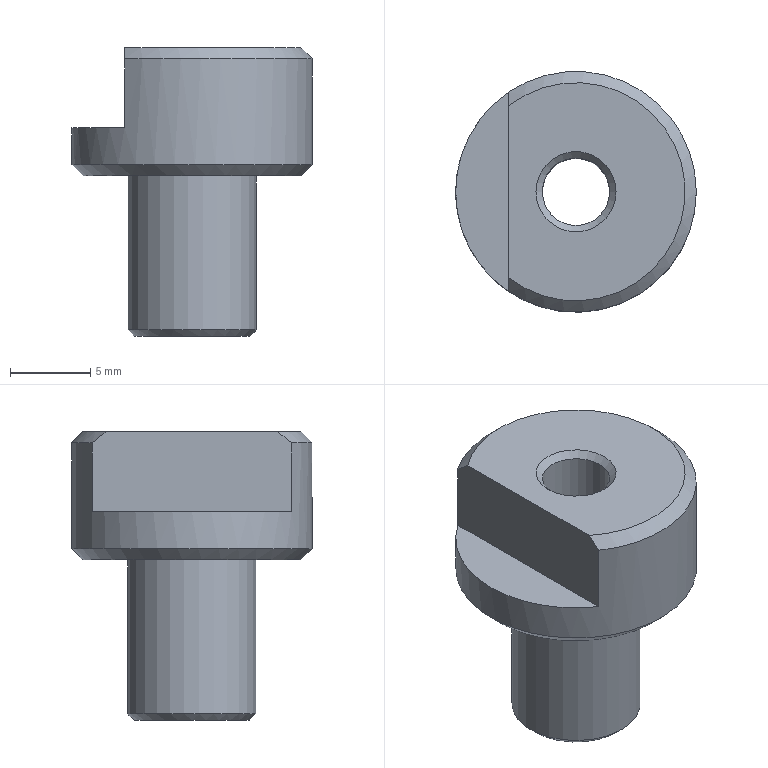Component | NX | DRILL_BUSHING_2 | 1 solid | 13 faces | box 15 x 15 x 18 mm | volume 1500 mm3 | plane 5 | cone 5 | cylinder 3 | commonest cylinder face diameters 8 x1 15 x1 4.2 x1
STEP:
#1=CARTESIAN_POINT('',(0.,0.,0.));
#2=DIRECTION('',(0.,0.,1.));
#3=DIRECTION('',(1.,0.,0.));
#4=AXIS2_PLACEMENT_3D('',#1,#2,#3);
#5=CARTESIAN_POINT('',(25.,0.,55.));
#6=VERTEX_POINT('',#5);
#7=CARTESIAN_POINT('',(22.5,0.,55.));
#8=DIRECTION('',(0.,0.,1.));
#9=DIRECTION('',(1.,0.,0.));
#10=AXIS2_PLACEMENT_3D('',#7,#8,#9);
#11=CIRCLE('',#10,2.5);
#12=CARTESIAN_POINT('',(22.5,0.,55.));
#13=DIRECTION('',(0.,0.,-1.));
#14=DIRECTION('',(1.,0.,0.));
#15=AXIS2_PLACEMENT_3D('',#12,#13,#14);
#16=PLANE('',#15);
#17=CARTESIAN_POINT('',(2.5,0.));
#18=CARTESIAN_POINT('',(2.5,-4.33));
#19=CARTESIAN_POINT('',(-1.25,-2.165));
#20=CARTESIAN_POINT('',(-5.,-0.));
#21=CARTESIAN_POINT('',(-1.25,2.165));
#22=CARTESIAN_POINT('',(2.5,4.33));
#23=CARTESIAN_POINT('',(2.5,0.));
#24=(BOUNDED_CURVE()B_SPLINE_CURVE(2,(#17,#18,#19,#20,#21,#22,#23),.UNSPECIFIED.,.T.,.F.)B_SPLINE_CURVE_WITH_KNOTS((1,2,2,2,2,1),(-2.094,0.,2.094,4.189,6.283,8.378),.UNSPECIFIED.)CURVE()GEOMETRIC_REPRESENTATION_ITEM()RATIONAL_B_SPLINE_CURVE((1.,0.5,1.,0.5,1.,0.5,1.))REPRESENTATION_ITEM(''));
#25=(GEOMETRIC_REPRESENTATION_CONTEXT(2)PARAMETRIC_REPRESENTATION_CONTEXT()REPRESENTATION_CONTEXT('',''));
#26=DEFINITIONAL_REPRESENTATION('',(#24),#25);
#27=PCURVE('',#16,#26);
#28=CARTESIAN_POINT('',(22.5,0.,55.4));
#29=DIRECTION('',(0.,0.,-1.));
#30=DIRECTION('',(1.,0.,0.));
#31=AXIS2_PLACEMENT_3D('',#28,#29,#30);
#32=CONICAL_SURFACE('',#31,2.1,0.7854);
#33=CARTESIAN_POINT('',(6.283,0.4));
#34=DIRECTION('',(-1.,0.));
#35=VECTOR('',#34,1.);
#36=LINE('',#33,#35);
#37=(GEOMETRIC_REPRESENTATION_CONTEXT(2)PARAMETRIC_REPRESENTATION_CONTEXT()REPRESENTATION_CONTEXT('',''));
#38=DEFINITIONAL_REPRESENTATION('',(#36),#37);
#39=PCURVE('',#32,#38);
#40=SURFACE_CURVE('',#11,(#27,#39),.PCURVE_S1.);
#41=EDGE_CURVE('',#6,#6,#40,.T.);
#42=ORIENTED_EDGE('',*,*,#41,.T.);
#43=EDGE_LOOP('',(#42));
#44=FACE_BOUND('',#43,.T.);
#45=CARTESIAN_POINT('',(26.1,0.,55.));
#46=VERTEX_POINT('',#45);
#47=CARTESIAN_POINT('',(22.5,0.,55.));
#48=DIRECTION('',(0.,0.,-1.));
#49=DIRECTION('',(1.,0.,0.));
#50=AXIS2_PLACEMENT_3D('',#47,#48,#49);
#51=CIRCLE('',#50,3.6);
#52=CARTESIAN_POINT('',(0.,0.));
#53=DIRECTION('',(1.,0.));
#54=AXIS2_PLACEMENT_2D('',#52,#53);
#55=CIRCLE('',#54,3.6);
#56=(GEOMETRIC_REPRESENTATION_CONTEXT(2)PARAMETRIC_REPRESENTATION_CONTEXT()REPRESENTATION_CONTEXT('',''));
#57=DEFINITIONAL_REPRESENTATION('',(#55),#56);
#58=PCURVE('',#16,#57);
#59=CARTESIAN_POINT('',(22.5,0.,55.4));
#60=DIRECTION('',(0.,0.,1.));
#61=DIRECTION('',(-1.,0.,0.));
#62=AXIS2_PLACEMENT_3D('',#59,#60,#61);
#63=CONICAL_SURFACE('',#62,4.,0.7854);
#64=CARTESIAN_POINT('',(9.425,-0.4));
#65=DIRECTION('',(-1.,0.));
#66=VECTOR('',#65,1.);
#67=LINE('',#64,#66);
#68=(GEOMETRIC_REPRESENTATION_CONTEXT(2)PARAMETRIC_REPRESENTATION_CONTEXT()REPRESENTATION_CONTEXT('',''));
#69=DEFINITIONAL_REPRESENTATION('',(#67),#68);
#70=PCURVE('',#63,#69);
#71=SURFACE_CURVE('',#51,(#58,#70),.PCURVE_S1.);
#72=EDGE_CURVE('',#46,#46,#71,.T.);
#73=ORIENTED_EDGE('',*,*,#72,.T.);
#74=EDGE_LOOP('',(#73));
#75=FACE_BOUND('',#74,.T.);
#76=ADVANCED_FACE('',(#44,#75),#16,.T.);
#77=CARTESIAN_POINT('',(26.5,0.,55.4));
#78=VERTEX_POINT('',#77);
#79=CARTESIAN_POINT('',(22.5,0.,55.4));
#80=DIRECTION('',(0.,0.,1.));
#81=DIRECTION('',(1.,0.,0.));
#82=AXIS2_PLACEMENT_3D('',#79,#80,#81);
#83=CIRCLE('',#82,4.);
#84=CARTESIAN_POINT('',(22.5,0.,55.));
#85=DIRECTION('',(0.,0.,1.));
#86=DIRECTION('',(-1.,0.,0.));
#87=AXIS2_PLACEMENT_3D('',#84,#85,#86);
#88=CYLINDRICAL_SURFACE('',#87,4.);
#89=CARTESIAN_POINT('',(3.142,0.4));
#90=DIRECTION('',(1.,0.));
#91=VECTOR('',#90,1.);
#92=LINE('',#89,#91);
#93=(GEOMETRIC_REPRESENTATION_CONTEXT(2)PARAMETRIC_REPRESENTATION_CONTEXT()REPRESENTATION_CONTEXT('',''));
#94=DEFINITIONAL_REPRESENTATION('',(#92),#93);
#95=PCURVE('',#88,#94);
#96=CARTESIAN_POINT('',(3.142,0.));
#97=DIRECTION('',(1.,0.));
#98=VECTOR('',#97,1.);
#99=LINE('',#96,#98);
#100=(GEOMETRIC_REPRESENTATION_CONTEXT(2)PARAMETRIC_REPRESENTATION_CONTEXT()REPRESENTATION_CONTEXT('',''));
#101=DEFINITIONAL_REPRESENTATION('',(#99),#100);
#102=PCURVE('',#63,#101);
#103=SURFACE_CURVE('',#83,(#95,#102),.PCURVE_S1.);
#104=EDGE_CURVE('',#78,#78,#103,.T.);
#105=ORIENTED_EDGE('',*,*,#104,.T.);
#106=CARTESIAN_POINT('',(26.5,0.,65.));
#107=VERTEX_POINT('',#106);
#108=CARTESIAN_POINT('',(26.5,0.,55.4));
#109=CARTESIAN_POINT('',(26.5,0.,65.));
#110=B_SPLINE_CURVE_WITH_KNOTS('',1,(#108,#109),.UNSPECIFIED.,.F.,.F.,(2,2),(0.4,10.),.PIECEWISE_BEZIER_KNOTS.);
#111=CARTESIAN_POINT('',(9.425,0.));
#112=DIRECTION('',(0.,1.));
#113=VECTOR('',#112,1.);
#114=LINE('',#111,#113);
#115=(GEOMETRIC_REPRESENTATION_CONTEXT(2)PARAMETRIC_REPRESENTATION_CONTEXT()REPRESENTATION_CONTEXT('',''));
#116=DEFINITIONAL_REPRESENTATION('',(#114),#115);
#117=PCURVE('',#88,#116);
#118=CARTESIAN_POINT('',(3.142,0.));
#119=DIRECTION('',(0.,1.));
#120=VECTOR('',#119,1.);
#121=LINE('',#118,#120);
#122=(GEOMETRIC_REPRESENTATION_CONTEXT(2)PARAMETRIC_REPRESENTATION_CONTEXT()REPRESENTATION_CONTEXT('',''));
#123=DEFINITIONAL_REPRESENTATION('',(#121),#122);
#124=PCURVE('',#88,#123);
#125=SEAM_CURVE('',#110,(#117,#124),.PCURVE_S1.);
#126=EDGE_CURVE('',#78,#107,#125,.T.);
#127=ORIENTED_EDGE('',*,*,#126,.T.);
#128=CARTESIAN_POINT('',(22.5,0.,65.));
#129=DIRECTION('',(0.,0.,1.));
#130=DIRECTION('',(1.,0.,0.));
#131=AXIS2_PLACEMENT_3D('',#128,#129,#130);
#132=CIRCLE('',#131,4.);
#133=CARTESIAN_POINT('',(3.142,10.));
#134=DIRECTION('',(1.,0.));
#135=VECTOR('',#134,1.);
#136=LINE('',#133,#135);
#137=(GEOMETRIC_REPRESENTATION_CONTEXT(2)PARAMETRIC_REPRESENTATION_CONTEXT()REPRESENTATION_CONTEXT('',''));
#138=DEFINITIONAL_REPRESENTATION('',(#136),#137);
#139=PCURVE('',#88,#138);
#140=CARTESIAN_POINT('',(22.5,0.,65.));
#141=DIRECTION('',(0.,0.,-1.));
#142=DIRECTION('',(1.,0.,0.));
#143=AXIS2_PLACEMENT_3D('',#140,#141,#142);
#144=PLANE('',#143);
#145=CARTESIAN_POINT('',(4.,0.));
#146=CARTESIAN_POINT('',(4.,-6.928));
#147=CARTESIAN_POINT('',(-2.,-3.464));
#148=CARTESIAN_POINT('',(-8.,-0.));
#149=CARTESIAN_POINT('',(-2.,3.464));
#150=CARTESIAN_POINT('',(4.,6.928));
#151=CARTESIAN_POINT('',(4.,0.));
#152=(BOUNDED_CURVE()B_SPLINE_CURVE(2,(#145,#146,#147,#148,#149,#150,#151),.UNSPECIFIED.,.T.,.F.)B_SPLINE_CURVE_WITH_KNOTS((1,2,2,2,2,1),(-2.094,0.,2.094,4.189,6.283,8.378),.UNSPECIFIED.)CURVE()GEOMETRIC_REPRESENTATION_ITEM()RATIONAL_B_SPLINE_CURVE((1.,0.5,1.,0.5,1.,0.5,1.))REPRESENTATION_ITEM(''));
#153=(GEOMETRIC_REPRESENTATION_CONTEXT(2)PARAMETRIC_REPRESENTATION_CONTEXT()REPRESENTATION_CONTEXT('',''));
#154=DEFINITIONAL_REPRESENTATION('',(#152),#153);
#155=PCURVE('',#144,#154);
#156=SURFACE_CURVE('',#132,(#139,#155),.PCURVE_S1.);
#157=EDGE_CURVE('',#107,#107,#156,.T.);
#158=ORIENTED_EDGE('',*,*,#157,.F.);
#159=ORIENTED_EDGE('',*,*,#126,.F.);
#160=EDGE_LOOP('',(#105,#127,#158,#159));
#161=FACE_BOUND('',#160,.T.);
#162=ADVANCED_FACE('',(#161),#88,.T.);
#163=CARTESIAN_POINT('',(20.,0.,73.));
#164=VERTEX_POINT('',#163);
#165=CARTESIAN_POINT('',(22.5,0.,73.));
#166=DIRECTION('',(0.,0.,-1.));
#167=DIRECTION('',(-1.,0.,0.));
#168=AXIS2_PLACEMENT_3D('',#165,#166,#167);
#169=CIRCLE('',#168,2.5);
#170=CARTESIAN_POINT('',(22.5,0.,73.));
#171=DIRECTION('',(0.,0.,1.));
#172=DIRECTION('',(-1.,0.,0.));
#173=AXIS2_PLACEMENT_3D('',#170,#171,#172);
#174=PLANE('',#173);
#175=CARTESIAN_POINT('',(2.5,0.));
#176=CARTESIAN_POINT('',(2.5,-4.33));
#177=CARTESIAN_POINT('',(-1.25,-2.165));
#178=CARTESIAN_POINT('',(-5.,-0.));
#179=CARTESIAN_POINT('',(-1.25,2.165));
#180=CARTESIAN_POINT('',(2.5,4.33));
#181=CARTESIAN_POINT('',(2.5,0.));
#182=(BOUNDED_CURVE()B_SPLINE_CURVE(2,(#175,#176,#177,#178,#179,#180,#181),.UNSPECIFIED.,.T.,.F.)B_SPLINE_CURVE_WITH_KNOTS((1,2,2,2,2,1),(-2.094,0.,2.094,4.189,6.283,8.378),.UNSPECIFIED.)CURVE()GEOMETRIC_REPRESENTATION_ITEM()RATIONAL_B_SPLINE_CURVE((1.,0.5,1.,0.5,1.,0.5,1.))REPRESENTATION_ITEM(''));
#183=(GEOMETRIC_REPRESENTATION_CONTEXT(2)PARAMETRIC_REPRESENTATION_CONTEXT()REPRESENTATION_CONTEXT('',''));
#184=DEFINITIONAL_REPRESENTATION('',(#182),#183);
#185=PCURVE('',#174,#184);
#186=CARTESIAN_POINT('',(22.5,0.,73.));
#187=DIRECTION('',(0.,0.,1.));
#188=DIRECTION('',(-1.,0.,0.));
#189=AXIS2_PLACEMENT_3D('',#186,#187,#188);
#190=CONICAL_SURFACE('',#189,2.5,0.7854);
#191=CARTESIAN_POINT('',(6.283,0.));
#192=DIRECTION('',(-1.,0.));
#193=VECTOR('',#192,1.);
#194=LINE('',#191,#193);
#195=(GEOMETRIC_REPRESENTATION_CONTEXT(2)PARAMETRIC_REPRESENTATION_CONTEXT()REPRESENTATION_CONTEXT('',''));
#196=DEFINITIONAL_REPRESENTATION('',(#194),#195);
#197=PCURVE('',#190,#196);
#198=SURFACE_CURVE('',#169,(#185,#197),.PCURVE_S1.);
#199=EDGE_CURVE('',#164,#164,#198,.T.);
#200=ORIENTED_EDGE('',*,*,#199,.T.);
#201=EDGE_LOOP('',(#200));
#202=FACE_BOUND('',#201,.T.);
#203=CARTESIAN_POINT('',(18.3,-5.348,73.));
#204=VERTEX_POINT('',#203);
#205=CARTESIAN_POINT('',(18.3,5.348,73.));
#206=VERTEX_POINT('',#205);
#207=CARTESIAN_POINT('',(18.3,-7.102,73.));
#208=DIRECTION('',(-0.,1.,0.));
#209=VECTOR('',#208,1.);
#210=LINE('',#207,#209);
#211=CARTESIAN_POINT('',(4.2,7.102));
#212=DIRECTION('',(0.,-1.));
#213=VECTOR('',#212,1.);
#214=LINE('',#211,#213);
#215=(GEOMETRIC_REPRESENTATION_CONTEXT(2)PARAMETRIC_REPRESENTATION_CONTEXT()REPRESENTATION_CONTEXT('',''));
#216=DEFINITIONAL_REPRESENTATION('',(#214),#215);
#217=PCURVE('',#174,#216);
#218=CARTESIAN_POINT('',(18.3,-7.102,68.));
#219=DIRECTION('',(1.,0.,0.));
#220=DIRECTION('',(-0.,1.,0.));
#221=AXIS2_PLACEMENT_3D('',#218,#219,#220);
#222=PLANE('',#221);
#223=CARTESIAN_POINT('',(0.,5.));
#224=DIRECTION('',(1.,0.));
#225=VECTOR('',#224,1.);
#226=LINE('',#223,#225);
#227=(GEOMETRIC_REPRESENTATION_CONTEXT(2)PARAMETRIC_REPRESENTATION_CONTEXT()REPRESENTATION_CONTEXT('',''));
#228=DEFINITIONAL_REPRESENTATION('',(#226),#227);
#229=PCURVE('',#222,#228);
#230=SURFACE_CURVE('',#210,(#217,#229),.PCURVE_S1.);
#231=EDGE_CURVE('',#204,#206,#230,.T.);
#232=ORIENTED_EDGE('',*,*,#231,.F.);
#233=CARTESIAN_POINT('',(22.5,0.,73.));
#234=DIRECTION('',(0.,0.,1.));
#235=DIRECTION('',(-1.,0.,0.));
#236=AXIS2_PLACEMENT_3D('',#233,#234,#235);
#237=CIRCLE('',#236,6.8);
#238=CARTESIAN_POINT('',(0.,0.));
#239=DIRECTION('',(1.,0.));
#240=AXIS2_PLACEMENT_2D('',#238,#239);
#241=CIRCLE('',#240,6.8);
#242=(GEOMETRIC_REPRESENTATION_CONTEXT(2)PARAMETRIC_REPRESENTATION_CONTEXT()REPRESENTATION_CONTEXT('',''));
#243=DEFINITIONAL_REPRESENTATION('',(#241),#242);
#244=PCURVE('',#174,#243);
#245=CARTESIAN_POINT('',(22.5,0.,72.3));
#246=DIRECTION('',(0.,0.,-1.));
#247=DIRECTION('',(1.,0.,0.));
#248=AXIS2_PLACEMENT_3D('',#245,#246,#247);
#249=CONICAL_SURFACE('',#248,7.5,0.7854);
#250=CARTESIAN_POINT('',(9.425,-0.7));
#251=DIRECTION('',(-1.,-0.));
#252=VECTOR('',#251,1.);
#253=LINE('',#250,#252);
#254=(GEOMETRIC_REPRESENTATION_CONTEXT(2)PARAMETRIC_REPRESENTATION_CONTEXT()REPRESENTATION_CONTEXT('',''));
#255=DEFINITIONAL_REPRESENTATION('',(#253),#254);
#256=PCURVE('',#249,#255);
#257=SURFACE_CURVE('',#237,(#244,#256),.PCURVE_S1.);
#258=EDGE_CURVE('',#204,#206,#257,.T.);
#259=ORIENTED_EDGE('',*,*,#258,.T.);
#260=EDGE_LOOP('',(#232,#259));
#261=FACE_BOUND('',#260,.T.);
#262=ADVANCED_FACE('',(#202,#261),#174,.T.);
#263=CARTESIAN_POINT('',(29.3,0.,65.));
#264=VERTEX_POINT('',#263);
#265=CARTESIAN_POINT('',(22.5,0.,65.));
#266=DIRECTION('',(0.,0.,-1.));
#267=DIRECTION('',(1.,0.,0.));
#268=AXIS2_PLACEMENT_3D('',#265,#266,#267);
#269=CIRCLE('',#268,6.8);
#270=CARTESIAN_POINT('',(0.,0.));
#271=DIRECTION('',(1.,0.));
#272=AXIS2_PLACEMENT_2D('',#270,#271);
#273=CIRCLE('',#272,6.8);
#274=(GEOMETRIC_REPRESENTATION_CONTEXT(2)PARAMETRIC_REPRESENTATION_CONTEXT()REPRESENTATION_CONTEXT('',''));
#275=DEFINITIONAL_REPRESENTATION('',(#273),#274);
#276=PCURVE('',#144,#275);
#277=CARTESIAN_POINT('',(22.5,0.,65.7));
#278=DIRECTION('',(0.,0.,1.));
#279=DIRECTION('',(-1.,0.,0.));
#280=AXIS2_PLACEMENT_3D('',#277,#278,#279);
#281=CONICAL_SURFACE('',#280,7.5,0.7854);
#282=CARTESIAN_POINT('',(9.425,-0.7));
#283=DIRECTION('',(-1.,0.));
#284=VECTOR('',#283,1.);
#285=LINE('',#282,#284);
#286=(GEOMETRIC_REPRESENTATION_CONTEXT(2)PARAMETRIC_REPRESENTATION_CONTEXT()REPRESENTATION_CONTEXT('',''));
#287=DEFINITIONAL_REPRESENTATION('',(#285),#286);
#288=PCURVE('',#281,#287);
#289=SURFACE_CURVE('',#269,(#276,#288),.PCURVE_S1.);
#290=EDGE_CURVE('',#264,#264,#289,.T.);
#291=ORIENTED_EDGE('',*,*,#290,.T.);
#292=EDGE_LOOP('',(#291));
#293=FACE_BOUND('',#292,.T.);
#294=ORIENTED_EDGE('',*,*,#157,.T.);
#295=EDGE_LOOP('',(#294));
#296=FACE_BOUND('',#295,.T.);
#297=ADVANCED_FACE('',(#293,#296),#144,.T.);
#298=CARTESIAN_POINT('',(30.,0.,65.7));
#299=VERTEX_POINT('',#298);
#300=CARTESIAN_POINT('',(18.3,6.214,65.7));
#301=VERTEX_POINT('',#300);
#302=CARTESIAN_POINT('',(22.5,0.,65.7));
#303=DIRECTION('',(0.,0.,1.));
#304=DIRECTION('',(1.,0.,0.));
#305=AXIS2_PLACEMENT_3D('',#302,#303,#304);
#306=CIRCLE('',#305,7.5);
#307=CARTESIAN_POINT('',(22.5,0.,65.));
#308=DIRECTION('',(0.,0.,1.));
#309=DIRECTION('',(-1.,0.,0.));
#310=AXIS2_PLACEMENT_3D('',#307,#308,#309);
#311=CYLINDRICAL_SURFACE('',#310,7.5);
#312=CARTESIAN_POINT('',(9.425,0.7));
#313=DIRECTION('',(1.,0.));
#314=VECTOR('',#313,1.);
#315=LINE('',#312,#314);
#316=(GEOMETRIC_REPRESENTATION_CONTEXT(2)PARAMETRIC_REPRESENTATION_CONTEXT()REPRESENTATION_CONTEXT('',''));
#317=DEFINITIONAL_REPRESENTATION('',(#315),#316);
#318=PCURVE('',#311,#317);
#319=CARTESIAN_POINT('',(3.142,0.));
#320=DIRECTION('',(1.,0.));
#321=VECTOR('',#320,1.);
#322=LINE('',#319,#321);
#323=(GEOMETRIC_REPRESENTATION_CONTEXT(2)PARAMETRIC_REPRESENTATION_CONTEXT()REPRESENTATION_CONTEXT('',''));
#324=DEFINITIONAL_REPRESENTATION('',(#322),#323);
#325=PCURVE('',#281,#324);
#326=SURFACE_CURVE('',#306,(#318,#325),.PCURVE_S1.);
#327=EDGE_CURVE('',#299,#301,#326,.T.);
#328=ORIENTED_EDGE('',*,*,#327,.T.);
#329=CARTESIAN_POINT('',(18.3,6.214,68.));
#330=VERTEX_POINT('',#329);
#331=CARTESIAN_POINT('',(18.3,6.214,65.7));
#332=CARTESIAN_POINT('',(18.3,6.214,68.));
#333=B_SPLINE_CURVE_WITH_KNOTS('',1,(#331,#332),.UNSPECIFIED.,.F.,.F.,(2,2),(0.7,3.),.PIECEWISE_BEZIER_KNOTS.);
#334=CARTESIAN_POINT('',(11.59,0.));
#335=DIRECTION('',(0.,1.));
#336=VECTOR('',#335,1.);
#337=LINE('',#334,#336);
#338=(GEOMETRIC_REPRESENTATION_CONTEXT(2)PARAMETRIC_REPRESENTATION_CONTEXT()REPRESENTATION_CONTEXT('',''));
#339=DEFINITIONAL_REPRESENTATION('',(#337),#338);
#340=PCURVE('',#311,#339);
#341=CARTESIAN_POINT('',(5.307,0.));
#342=DIRECTION('',(0.,1.));
#343=VECTOR('',#342,1.);
#344=LINE('',#341,#343);
#345=(GEOMETRIC_REPRESENTATION_CONTEXT(2)PARAMETRIC_REPRESENTATION_CONTEXT()REPRESENTATION_CONTEXT('',''));
#346=DEFINITIONAL_REPRESENTATION('',(#344),#345);
#347=PCURVE('',#311,#346);
#348=SEAM_CURVE('',#333,(#340,#347),.PCURVE_S1.);
#349=EDGE_CURVE('',#301,#330,#348,.T.);
#350=ORIENTED_EDGE('',*,*,#349,.T.);
#351=CARTESIAN_POINT('',(18.3,6.214,72.3));
#352=VERTEX_POINT('',#351);
#353=CARTESIAN_POINT('',(18.3,6.214,65.));
#354=DIRECTION('',(0.,0.,-1.));
#355=VECTOR('',#354,1.);
#356=LINE('',#353,#355);
#357=CARTESIAN_POINT('',(11.59,0.));
#358=DIRECTION('',(0.,-1.));
#359=VECTOR('',#358,1.);
#360=LINE('',#357,#359);
#361=(GEOMETRIC_REPRESENTATION_CONTEXT(2)PARAMETRIC_REPRESENTATION_CONTEXT()REPRESENTATION_CONTEXT('',''));
#362=DEFINITIONAL_REPRESENTATION('',(#360),#361);
#363=PCURVE('',#311,#362);
#364=CARTESIAN_POINT('',(13.316,-3.));
#365=DIRECTION('',(0.,-1.));
#366=VECTOR('',#365,1.);
#367=LINE('',#364,#366);
#368=(GEOMETRIC_REPRESENTATION_CONTEXT(2)PARAMETRIC_REPRESENTATION_CONTEXT()REPRESENTATION_CONTEXT('',''));
#369=DEFINITIONAL_REPRESENTATION('',(#367),#368);
#370=PCURVE('',#222,#369);
#371=SURFACE_CURVE('',#356,(#363,#370),.PCURVE_S1.);
#372=EDGE_CURVE('',#352,#330,#371,.T.);
#373=ORIENTED_EDGE('',*,*,#372,.F.);
#374=CARTESIAN_POINT('',(18.3,-6.214,72.3));
#375=VERTEX_POINT('',#374);
#376=CARTESIAN_POINT('',(22.5,0.,72.3));
#377=DIRECTION('',(0.,0.,-1.));
#378=DIRECTION('',(-1.,0.,0.));
#379=AXIS2_PLACEMENT_3D('',#376,#377,#378);
#380=CIRCLE('',#379,7.5);
#381=CARTESIAN_POINT('',(12.566,7.3));
#382=DIRECTION('',(-1.,0.));
#383=VECTOR('',#382,1.);
#384=LINE('',#381,#383);
#385=(GEOMETRIC_REPRESENTATION_CONTEXT(2)PARAMETRIC_REPRESENTATION_CONTEXT()REPRESENTATION_CONTEXT('',''));
#386=DEFINITIONAL_REPRESENTATION('',(#384),#385);
#387=PCURVE('',#311,#386);
#388=CARTESIAN_POINT('',(3.142,0.));
#389=DIRECTION('',(1.,-0.));
#390=VECTOR('',#389,1.);
#391=LINE('',#388,#390);
#392=(GEOMETRIC_REPRESENTATION_CONTEXT(2)PARAMETRIC_REPRESENTATION_CONTEXT()REPRESENTATION_CONTEXT('',''));
#393=DEFINITIONAL_REPRESENTATION('',(#391),#392);
#394=PCURVE('',#249,#393);
#395=SURFACE_CURVE('',#380,(#387,#394),.PCURVE_S1.);
#396=EDGE_CURVE('',#352,#375,#395,.T.);
#397=ORIENTED_EDGE('',*,*,#396,.T.);
#398=CARTESIAN_POINT('',(18.3,-6.214,68.));
#399=VERTEX_POINT('',#398);
#400=CARTESIAN_POINT('',(18.3,-6.214,65.));
#401=DIRECTION('',(0.,0.,1.));
#402=VECTOR('',#401,1.);
#403=LINE('',#400,#402);
#404=CARTESIAN_POINT('',(7.26,0.));
#405=DIRECTION('',(0.,1.));
#406=VECTOR('',#405,1.);
#407=LINE('',#404,#406);
#408=(GEOMETRIC_REPRESENTATION_CONTEXT(2)PARAMETRIC_REPRESENTATION_CONTEXT()REPRESENTATION_CONTEXT('',''));
#409=DEFINITIONAL_REPRESENTATION('',(#407),#408);
#410=PCURVE('',#311,#409);
#411=CARTESIAN_POINT('',(0.8883,-3.));
#412=DIRECTION('',(0.,1.));
#413=VECTOR('',#412,1.);
#414=LINE('',#411,#413);
#415=(GEOMETRIC_REPRESENTATION_CONTEXT(2)PARAMETRIC_REPRESENTATION_CONTEXT()REPRESENTATION_CONTEXT('',''));
#416=DEFINITIONAL_REPRESENTATION('',(#414),#415);
#417=PCURVE('',#222,#416);
#418=SURFACE_CURVE('',#403,(#410,#417),.PCURVE_S1.);
#419=EDGE_CURVE('',#399,#375,#418,.T.);
#420=ORIENTED_EDGE('',*,*,#419,.F.);
#421=CARTESIAN_POINT('',(22.5,0.,68.));
#422=DIRECTION('',(0.,0.,-1.));
#423=DIRECTION('',(-1.,0.,0.));
#424=AXIS2_PLACEMENT_3D('',#421,#422,#423);
#425=CIRCLE('',#424,7.5);
#426=CARTESIAN_POINT('',(12.566,3.));
#427=DIRECTION('',(-1.,0.));
#428=VECTOR('',#427,1.);
#429=LINE('',#426,#428);
#430=(GEOMETRIC_REPRESENTATION_CONTEXT(2)PARAMETRIC_REPRESENTATION_CONTEXT()REPRESENTATION_CONTEXT('',''));
#431=DEFINITIONAL_REPRESENTATION('',(#429),#430);
#432=PCURVE('',#311,#431);
#433=CARTESIAN_POINT('',(22.5,0.,68.));
#434=DIRECTION('',(0.,0.,1.));
#435=DIRECTION('',(-1.,0.,0.));
#436=AXIS2_PLACEMENT_3D('',#433,#434,#435);
#437=PLANE('',#436);
#438=CARTESIAN_POINT('',(7.5,0.));
#439=CARTESIAN_POINT('',(7.5,-12.99));
#440=CARTESIAN_POINT('',(-3.75,-6.495));
#441=CARTESIAN_POINT('',(-15.,-0.));
#442=CARTESIAN_POINT('',(-3.75,6.495));
#443=CARTESIAN_POINT('',(7.5,12.99));
#444=CARTESIAN_POINT('',(7.5,0.));
#445=(BOUNDED_CURVE()B_SPLINE_CURVE(2,(#438,#439,#440,#441,#442,#443,#444),.UNSPECIFIED.,.T.,.F.)B_SPLINE_CURVE_WITH_KNOTS((1,2,2,2,2,1),(-2.094,0.,2.094,4.189,6.283,8.378),.UNSPECIFIED.)CURVE()GEOMETRIC_REPRESENTATION_ITEM()RATIONAL_B_SPLINE_CURVE((1.,0.5,1.,0.5,1.,0.5,1.))REPRESENTATION_ITEM(''));
#446=(GEOMETRIC_REPRESENTATION_CONTEXT(2)PARAMETRIC_REPRESENTATION_CONTEXT()REPRESENTATION_CONTEXT('',''));
#447=DEFINITIONAL_REPRESENTATION('',(#445),#446);
#448=PCURVE('',#437,#447);
#449=SURFACE_CURVE('',#425,(#432,#448),.PCURVE_S1.);
#450=EDGE_CURVE('',#399,#330,#449,.T.);
#451=ORIENTED_EDGE('',*,*,#450,.T.);
#452=ORIENTED_EDGE('',*,*,#349,.F.);
#453=CARTESIAN_POINT('',(22.5,0.,65.7));
#454=DIRECTION('',(0.,0.,1.));
#455=DIRECTION('',(1.,0.,0.));
#456=AXIS2_PLACEMENT_3D('',#453,#454,#455);
#457=CIRCLE('',#456,7.5);
#458=CARTESIAN_POINT('',(3.142,0.7));
#459=DIRECTION('',(1.,0.));
#460=VECTOR('',#459,1.);
#461=LINE('',#458,#460);
#462=(GEOMETRIC_REPRESENTATION_CONTEXT(2)PARAMETRIC_REPRESENTATION_CONTEXT()REPRESENTATION_CONTEXT('',''));
#463=DEFINITIONAL_REPRESENTATION('',(#461),#462);
#464=PCURVE('',#311,#463);
#465=CARTESIAN_POINT('',(3.142,0.));
#466=DIRECTION('',(1.,0.));
#467=VECTOR('',#466,1.);
#468=LINE('',#465,#467);
#469=(GEOMETRIC_REPRESENTATION_CONTEXT(2)PARAMETRIC_REPRESENTATION_CONTEXT()REPRESENTATION_CONTEXT('',''));
#470=DEFINITIONAL_REPRESENTATION('',(#468),#469);
#471=PCURVE('',#281,#470);
#472=SURFACE_CURVE('',#457,(#464,#471),.PCURVE_S1.);
#473=EDGE_CURVE('',#301,#299,#472,.T.);
#474=ORIENTED_EDGE('',*,*,#473,.T.);
#475=EDGE_LOOP('',(#328,#350,#373,#397,#420,#451,#452,#474));
#476=FACE_BOUND('',#475,.T.);
#477=ADVANCED_FACE('',(#476),#311,.T.);
#478=CARTESIAN_POINT('',(24.6,0.,72.6));
#479=VERTEX_POINT('',#478);
#480=CARTESIAN_POINT('',(20.4,0.,72.6));
#481=VERTEX_POINT('',#480);
#482=CARTESIAN_POINT('',(22.5,0.,72.6));
#483=DIRECTION('',(0.,0.,1.));
#484=DIRECTION('',(-1.,0.,0.));
#485=AXIS2_PLACEMENT_3D('',#482,#483,#484);
#486=CIRCLE('',#485,2.1);
#487=CARTESIAN_POINT('',(22.5,0.,73.));
#488=DIRECTION('',(0.,0.,-1.));
#489=DIRECTION('',(1.,0.,0.));
#490=AXIS2_PLACEMENT_3D('',#487,#488,#489);
#491=CYLINDRICAL_SURFACE('',#490,2.1);
#492=CARTESIAN_POINT('',(9.425,0.4));
#493=DIRECTION('',(-1.,0.));
#494=VECTOR('',#493,1.);
#495=LINE('',#492,#494);
#496=(GEOMETRIC_REPRESENTATION_CONTEXT(2)PARAMETRIC_REPRESENTATION_CONTEXT()REPRESENTATION_CONTEXT('',''));
#497=DEFINITIONAL_REPRESENTATION('',(#495),#496);
#498=PCURVE('',#491,#497);
#499=CARTESIAN_POINT('',(0.,-0.4));
#500=DIRECTION('',(1.,0.));
#501=VECTOR('',#500,1.);
#502=LINE('',#499,#501);
#503=(GEOMETRIC_REPRESENTATION_CONTEXT(2)PARAMETRIC_REPRESENTATION_CONTEXT()REPRESENTATION_CONTEXT('',''));
#504=DEFINITIONAL_REPRESENTATION('',(#502),#503);
#505=PCURVE('',#190,#504);
#506=SURFACE_CURVE('',#486,(#498,#505),.PCURVE_S1.);
#507=EDGE_CURVE('',#479,#481,#506,.T.);
#508=ORIENTED_EDGE('',*,*,#507,.F.);
#509=CARTESIAN_POINT('',(24.6,0.,55.4));
#510=VERTEX_POINT('',#509);
#511=CARTESIAN_POINT('',(24.6,0.,72.6));
#512=CARTESIAN_POINT('',(24.6,0.,55.4));
#513=B_SPLINE_CURVE_WITH_KNOTS('',1,(#511,#512),.UNSPECIFIED.,.F.,.F.,(2,2),(0.4,17.6),.PIECEWISE_BEZIER_KNOTS.);
#514=CARTESIAN_POINT('',(6.283,0.));
#515=DIRECTION('',(0.,1.));
#516=VECTOR('',#515,1.);
#517=LINE('',#514,#516);
#518=(GEOMETRIC_REPRESENTATION_CONTEXT(2)PARAMETRIC_REPRESENTATION_CONTEXT()REPRESENTATION_CONTEXT('',''));
#519=DEFINITIONAL_REPRESENTATION('',(#517),#518);
#520=PCURVE('',#491,#519);
#521=CARTESIAN_POINT('',(0.,0.));
#522=DIRECTION('',(0.,1.));
#523=VECTOR('',#522,1.);
#524=LINE('',#521,#523);
#525=(GEOMETRIC_REPRESENTATION_CONTEXT(2)PARAMETRIC_REPRESENTATION_CONTEXT()REPRESENTATION_CONTEXT('',''));
#526=DEFINITIONAL_REPRESENTATION('',(#524),#525);
#527=PCURVE('',#491,#526);
#528=SEAM_CURVE('',#513,(#520,#527),.PCURVE_S1.);
#529=EDGE_CURVE('',#479,#510,#528,.T.);
#530=ORIENTED_EDGE('',*,*,#529,.T.);
#531=CARTESIAN_POINT('',(22.5,0.,55.4));
#532=DIRECTION('',(0.,0.,-1.));
#533=DIRECTION('',(1.,0.,0.));
#534=AXIS2_PLACEMENT_3D('',#531,#532,#533);
#535=CIRCLE('',#534,2.1);
#536=CARTESIAN_POINT('',(0.,17.6));
#537=DIRECTION('',(1.,0.));
#538=VECTOR('',#537,1.);
#539=LINE('',#536,#538);
#540=(GEOMETRIC_REPRESENTATION_CONTEXT(2)PARAMETRIC_REPRESENTATION_CONTEXT()REPRESENTATION_CONTEXT('',''));
#541=DEFINITIONAL_REPRESENTATION('',(#539),#540);
#542=PCURVE('',#491,#541);
#543=CARTESIAN_POINT('',(0.,0.));
#544=DIRECTION('',(1.,0.));
#545=VECTOR('',#544,1.);
#546=LINE('',#543,#545);
#547=(GEOMETRIC_REPRESENTATION_CONTEXT(2)PARAMETRIC_REPRESENTATION_CONTEXT()REPRESENTATION_CONTEXT('',''));
#548=DEFINITIONAL_REPRESENTATION('',(#546),#547);
#549=PCURVE('',#32,#548);
#550=SURFACE_CURVE('',#535,(#542,#549),.PCURVE_S1.);
#551=EDGE_CURVE('',#510,#510,#550,.T.);
#552=ORIENTED_EDGE('',*,*,#551,.F.);
#553=ORIENTED_EDGE('',*,*,#529,.F.);
#554=CARTESIAN_POINT('',(22.5,0.,72.6));
#555=DIRECTION('',(0.,0.,1.));
#556=DIRECTION('',(-1.,0.,0.));
#557=AXIS2_PLACEMENT_3D('',#554,#555,#556);
#558=CIRCLE('',#557,2.1);
#559=CARTESIAN_POINT('',(3.142,0.4));
#560=DIRECTION('',(-1.,0.));
#561=VECTOR('',#560,1.);
#562=LINE('',#559,#561);
#563=(GEOMETRIC_REPRESENTATION_CONTEXT(2)PARAMETRIC_REPRESENTATION_CONTEXT()REPRESENTATION_CONTEXT('',''));
#564=DEFINITIONAL_REPRESENTATION('',(#562),#563);
#565=PCURVE('',#491,#564);
#566=CARTESIAN_POINT('',(0.,-0.4));
#567=DIRECTION('',(1.,0.));
#568=VECTOR('',#567,1.);
#569=LINE('',#566,#568);
#570=(GEOMETRIC_REPRESENTATION_CONTEXT(2)PARAMETRIC_REPRESENTATION_CONTEXT()REPRESENTATION_CONTEXT('',''));
#571=DEFINITIONAL_REPRESENTATION('',(#569),#570);
#572=PCURVE('',#190,#571);
#573=SURFACE_CURVE('',#558,(#565,#572),.PCURVE_S1.);
#574=EDGE_CURVE('',#481,#479,#573,.T.);
#575=ORIENTED_EDGE('',*,*,#574,.F.);
#576=EDGE_LOOP('',(#508,#530,#552,#553,#575));
#577=FACE_BOUND('',#576,.F.);
#578=ADVANCED_FACE('',(#577),#491,.F.);
#579=ORIENTED_EDGE('',*,*,#419,.T.);
#580=CARTESIAN_POINT('',(18.3,-6.214,72.3));
#581=CARTESIAN_POINT('',(18.3,-5.928,72.537));
#582=CARTESIAN_POINT('',(18.3,-5.64,72.771));
#583=CARTESIAN_POINT('',(18.3,-5.348,73.));
#584=B_SPLINE_CURVE_WITH_KNOTS('',3,(#580,#581,#582,#583),.UNSPECIFIED.,.F.,.F.,(4,4),(0.,1.),.PIECEWISE_BEZIER_KNOTS.);
#585=CARTESIAN_POINT('',(0.8883,4.3));
#586=CARTESIAN_POINT('',(1.174,4.537));
#587=CARTESIAN_POINT('',(1.462,4.771));
#588=CARTESIAN_POINT('',(1.754,5.));
#589=B_SPLINE_CURVE_WITH_KNOTS('',3,(#585,#586,#587,#588),.UNSPECIFIED.,.F.,.F.,(4,4),(0.,1.),.PIECEWISE_BEZIER_KNOTS.);
#590=(GEOMETRIC_REPRESENTATION_CONTEXT(2)PARAMETRIC_REPRESENTATION_CONTEXT()REPRESENTATION_CONTEXT('',''));
#591=DEFINITIONAL_REPRESENTATION('',(#589),#590);
#592=PCURVE('',#222,#591);
#593=CARTESIAN_POINT('',(8.448,-0.));
#594=CARTESIAN_POINT('',(8.52,-0.7));
#595=B_SPLINE_CURVE_WITH_KNOTS('',1,(#593,#594),.UNSPECIFIED.,.F.,.F.,(2,2),(0.,1.),.PIECEWISE_BEZIER_KNOTS.);
#596=(GEOMETRIC_REPRESENTATION_CONTEXT(2)PARAMETRIC_REPRESENTATION_CONTEXT()REPRESENTATION_CONTEXT('',''));
#597=DEFINITIONAL_REPRESENTATION('',(#595),#596);
#598=PCURVE('',#249,#597);
#599=SURFACE_CURVE('',#584,(#592,#598),.PCURVE_S1.);
#600=EDGE_CURVE('',#375,#204,#599,.T.);
#601=ORIENTED_EDGE('',*,*,#600,.T.);
#602=ORIENTED_EDGE('',*,*,#231,.T.);
#603=CARTESIAN_POINT('',(18.3,5.348,73.));
#604=CARTESIAN_POINT('',(18.3,5.64,72.771));
#605=CARTESIAN_POINT('',(18.3,5.928,72.537));
#606=CARTESIAN_POINT('',(18.3,6.214,72.3));
#607=B_SPLINE_CURVE_WITH_KNOTS('',3,(#603,#604,#605,#606),.UNSPECIFIED.,.F.,.F.,(4,4),(0.,1.),.PIECEWISE_BEZIER_KNOTS.);
#608=CARTESIAN_POINT('',(12.45,5.));
#609=CARTESIAN_POINT('',(12.742,4.771));
#610=CARTESIAN_POINT('',(13.03,4.537));
#611=CARTESIAN_POINT('',(13.316,4.3));
#612=B_SPLINE_CURVE_WITH_KNOTS('',3,(#608,#609,#610,#611),.UNSPECIFIED.,.F.,.F.,(4,4),(0.,1.),.PIECEWISE_BEZIER_KNOTS.);
#613=(GEOMETRIC_REPRESENTATION_CONTEXT(2)PARAMETRIC_REPRESENTATION_CONTEXT()REPRESENTATION_CONTEXT('',''));
#614=DEFINITIONAL_REPRESENTATION('',(#612),#613);
#615=PCURVE('',#222,#614);
#616=CARTESIAN_POINT('',(4.047,-0.7));
#617=CARTESIAN_POINT('',(4.118,-0.));
#618=B_SPLINE_CURVE_WITH_KNOTS('',1,(#616,#617),.UNSPECIFIED.,.F.,.F.,(2,2),(0.,1.),.PIECEWISE_BEZIER_KNOTS.);
#619=(GEOMETRIC_REPRESENTATION_CONTEXT(2)PARAMETRIC_REPRESENTATION_CONTEXT()REPRESENTATION_CONTEXT('',''));
#620=DEFINITIONAL_REPRESENTATION('',(#618),#619);
#621=PCURVE('',#249,#620);
#622=SURFACE_CURVE('',#607,(#615,#621),.PCURVE_S1.);
#623=EDGE_CURVE('',#206,#352,#622,.T.);
#624=ORIENTED_EDGE('',*,*,#623,.T.);
#625=ORIENTED_EDGE('',*,*,#372,.T.);
#626=CARTESIAN_POINT('',(18.3,-7.102,68.));
#627=DIRECTION('',(0.,-1.,0.));
#628=VECTOR('',#627,1.);
#629=LINE('',#626,#628);
#630=CARTESIAN_POINT('',(0.,0.));
#631=DIRECTION('',(-1.,0.));
#632=VECTOR('',#631,1.);
#633=LINE('',#630,#632);
#634=(GEOMETRIC_REPRESENTATION_CONTEXT(2)PARAMETRIC_REPRESENTATION_CONTEXT()REPRESENTATION_CONTEXT('',''));
#635=DEFINITIONAL_REPRESENTATION('',(#633),#634);
#636=PCURVE('',#222,#635);
#637=CARTESIAN_POINT('',(4.2,7.102));
#638=DIRECTION('',(-0.,1.));
#639=VECTOR('',#638,1.);
#640=LINE('',#637,#639);
#641=(GEOMETRIC_REPRESENTATION_CONTEXT(2)PARAMETRIC_REPRESENTATION_CONTEXT()REPRESENTATION_CONTEXT('',''));
#642=DEFINITIONAL_REPRESENTATION('',(#640),#641);
#643=PCURVE('',#437,#642);
#644=SURFACE_CURVE('',#629,(#636,#643),.PCURVE_S1.);
#645=EDGE_CURVE('',#330,#399,#644,.T.);
#646=ORIENTED_EDGE('',*,*,#645,.T.);
#647=EDGE_LOOP('',(#579,#601,#602,#624,#625,#646));
#648=FACE_BOUND('',#647,.T.);
#649=ADVANCED_FACE('',(#648),#222,.F.);
#650=ORIENTED_EDGE('',*,*,#645,.F.);
#651=ORIENTED_EDGE('',*,*,#450,.F.);
#652=EDGE_LOOP('',(#650,#651));
#653=FACE_BOUND('',#652,.T.);
#654=ADVANCED_FACE('',(#653),#437,.T.);
#655=ORIENTED_EDGE('',*,*,#290,.F.);
#656=CARTESIAN_POINT('',(29.3,0.,65.));
#657=CARTESIAN_POINT('',(30.,0.,65.7));
#658=B_SPLINE_CURVE_WITH_KNOTS('',1,(#656,#657),.UNSPECIFIED.,.F.,.F.,(2,2),(-0.9899,0.),.PIECEWISE_BEZIER_KNOTS.);
#659=CARTESIAN_POINT('',(9.425,0.));
#660=DIRECTION('',(0.,1.));
#661=VECTOR('',#660,1.);
#662=LINE('',#659,#661);
#663=(GEOMETRIC_REPRESENTATION_CONTEXT(2)PARAMETRIC_REPRESENTATION_CONTEXT()REPRESENTATION_CONTEXT('',''));
#664=DEFINITIONAL_REPRESENTATION('',(#662),#663);
#665=PCURVE('',#281,#664);
#666=CARTESIAN_POINT('',(3.142,0.));
#667=DIRECTION('',(0.,1.));
#668=VECTOR('',#667,1.);
#669=LINE('',#666,#668);
#670=(GEOMETRIC_REPRESENTATION_CONTEXT(2)PARAMETRIC_REPRESENTATION_CONTEXT()REPRESENTATION_CONTEXT('',''));
#671=DEFINITIONAL_REPRESENTATION('',(#669),#670);
#672=PCURVE('',#281,#671);
#673=SEAM_CURVE('',#658,(#665,#672),.PCURVE_S1.);
#674=EDGE_CURVE('',#264,#299,#673,.T.);
#675=ORIENTED_EDGE('',*,*,#674,.T.);
#676=ORIENTED_EDGE('',*,*,#473,.F.);
#677=ORIENTED_EDGE('',*,*,#327,.F.);
#678=ORIENTED_EDGE('',*,*,#674,.F.);
#679=EDGE_LOOP('',(#655,#675,#676,#677,#678));
#680=FACE_BOUND('',#679,.T.);
#681=ADVANCED_FACE('',(#680),#281,.T.);
#682=ORIENTED_EDGE('',*,*,#623,.F.);
#683=ORIENTED_EDGE('',*,*,#258,.F.);
#684=ORIENTED_EDGE('',*,*,#600,.F.);
#685=ORIENTED_EDGE('',*,*,#396,.F.);
#686=EDGE_LOOP('',(#682,#683,#684,#685));
#687=FACE_BOUND('',#686,.T.);
#688=ADVANCED_FACE('',(#687),#249,.T.);
#689=ORIENTED_EDGE('',*,*,#507,.T.);
#690=CARTESIAN_POINT('',(20.4,0.,72.6));
#691=CARTESIAN_POINT('',(20.,0.,73.));
#692=B_SPLINE_CURVE_WITH_KNOTS('',1,(#690,#691),.UNSPECIFIED.,.F.,.F.,(2,2),(-0.5657,0.),.PIECEWISE_BEZIER_KNOTS.);
#693=CARTESIAN_POINT('',(6.283,0.));
#694=DIRECTION('',(0.,1.));
#695=VECTOR('',#694,1.);
#696=LINE('',#693,#695);
#697=(GEOMETRIC_REPRESENTATION_CONTEXT(2)PARAMETRIC_REPRESENTATION_CONTEXT()REPRESENTATION_CONTEXT('',''));
#698=DEFINITIONAL_REPRESENTATION('',(#696),#697);
#699=PCURVE('',#190,#698);
#700=CARTESIAN_POINT('',(0.,0.));
#701=DIRECTION('',(0.,1.));
#702=VECTOR('',#701,1.);
#703=LINE('',#700,#702);
#704=(GEOMETRIC_REPRESENTATION_CONTEXT(2)PARAMETRIC_REPRESENTATION_CONTEXT()REPRESENTATION_CONTEXT('',''));
#705=DEFINITIONAL_REPRESENTATION('',(#703),#704);
#706=PCURVE('',#190,#705);
#707=SEAM_CURVE('',#692,(#699,#706),.PCURVE_S1.);
#708=EDGE_CURVE('',#481,#164,#707,.T.);
#709=ORIENTED_EDGE('',*,*,#708,.T.);
#710=ORIENTED_EDGE('',*,*,#199,.T.);
#711=ORIENTED_EDGE('',*,*,#708,.F.);
#712=ORIENTED_EDGE('',*,*,#574,.T.);
#713=EDGE_LOOP('',(#689,#709,#710,#711,#712));
#714=FACE_BOUND('',#713,.F.);
#715=ADVANCED_FACE('',(#714),#190,.F.);
#716=ORIENTED_EDGE('',*,*,#41,.T.);
#717=CARTESIAN_POINT('',(24.6,0.,55.4));
#718=CARTESIAN_POINT('',(25.,0.,55.));
#719=B_SPLINE_CURVE_WITH_KNOTS('',1,(#717,#718),.UNSPECIFIED.,.F.,.F.,(2,2),(0.,0.5657),.PIECEWISE_BEZIER_KNOTS.);
#720=CARTESIAN_POINT('',(0.,0.));
#721=DIRECTION('',(0.,1.));
#722=VECTOR('',#721,1.);
#723=LINE('',#720,#722);
#724=(GEOMETRIC_REPRESENTATION_CONTEXT(2)PARAMETRIC_REPRESENTATION_CONTEXT()REPRESENTATION_CONTEXT('',''));
#725=DEFINITIONAL_REPRESENTATION('',(#723),#724);
#726=PCURVE('',#32,#725);
#727=CARTESIAN_POINT('',(6.283,0.));
#728=DIRECTION('',(0.,1.));
#729=VECTOR('',#728,1.);
#730=LINE('',#727,#729);
#731=(GEOMETRIC_REPRESENTATION_CONTEXT(2)PARAMETRIC_REPRESENTATION_CONTEXT()REPRESENTATION_CONTEXT('',''));
#732=DEFINITIONAL_REPRESENTATION('',(#730),#731);
#733=PCURVE('',#32,#732);
#734=SEAM_CURVE('',#719,(#726,#733),.PCURVE_S1.);
#735=EDGE_CURVE('',#510,#6,#734,.T.);
#736=ORIENTED_EDGE('',*,*,#735,.F.);
#737=ORIENTED_EDGE('',*,*,#551,.T.);
#738=ORIENTED_EDGE('',*,*,#735,.T.);
#739=EDGE_LOOP('',(#716,#736,#737,#738));
#740=FACE_BOUND('',#739,.F.);
#741=ADVANCED_FACE('',(#740),#32,.F.);
#742=ORIENTED_EDGE('',*,*,#72,.F.);
#743=CARTESIAN_POINT('',(26.1,0.,55.));
#744=CARTESIAN_POINT('',(26.5,0.,55.4));
#745=B_SPLINE_CURVE_WITH_KNOTS('',1,(#743,#744),.UNSPECIFIED.,.F.,.F.,(2,2),(-0.5657,0.),.PIECEWISE_BEZIER_KNOTS.);
#746=CARTESIAN_POINT('',(9.425,0.));
#747=DIRECTION('',(0.,1.));
#748=VECTOR('',#747,1.);
#749=LINE('',#746,#748);
#750=(GEOMETRIC_REPRESENTATION_CONTEXT(2)PARAMETRIC_REPRESENTATION_CONTEXT()REPRESENTATION_CONTEXT('',''));
#751=DEFINITIONAL_REPRESENTATION('',(#749),#750);
#752=PCURVE('',#63,#751);
#753=CARTESIAN_POINT('',(3.142,0.));
#754=DIRECTION('',(0.,1.));
#755=VECTOR('',#754,1.);
#756=LINE('',#753,#755);
#757=(GEOMETRIC_REPRESENTATION_CONTEXT(2)PARAMETRIC_REPRESENTATION_CONTEXT()REPRESENTATION_CONTEXT('',''));
#758=DEFINITIONAL_REPRESENTATION('',(#756),#757);
#759=PCURVE('',#63,#758);
#760=SEAM_CURVE('',#745,(#752,#759),.PCURVE_S1.);
#761=EDGE_CURVE('',#46,#78,#760,.T.);
#762=ORIENTED_EDGE('',*,*,#761,.T.);
#763=ORIENTED_EDGE('',*,*,#104,.F.);
#764=ORIENTED_EDGE('',*,*,#761,.F.);
#765=EDGE_LOOP('',(#742,#762,#763,#764));
#766=FACE_BOUND('',#765,.T.);
#767=ADVANCED_FACE('',(#766),#63,.T.);
#768=CLOSED_SHELL('',(#76,#162,#262,#297,#477,#578,#649,#654,#681,#688,#715,#741,#767));
#769=MANIFOLD_SOLID_BREP('',#768);
#770=(LENGTH_UNIT()NAMED_UNIT(*)SI_UNIT(.MILLI.,.METRE.));
#771=UNCERTAINTY_MEASURE_WITH_UNIT(LENGTH_MEASURE(0.002),#770,'','');
#772=(NAMED_UNIT(*)PLANE_ANGLE_UNIT()SI_UNIT($,.RADIAN.));
#773=(NAMED_UNIT(*)SI_UNIT($,.STERADIAN.)SOLID_ANGLE_UNIT());
#774=(GEOMETRIC_REPRESENTATION_CONTEXT(3)GLOBAL_UNCERTAINTY_ASSIGNED_CONTEXT((#771))GLOBAL_UNIT_ASSIGNED_CONTEXT((#770,#772,#773))REPRESENTATION_CONTEXT('',''));
#775=ADVANCED_BREP_SHAPE_REPRESENTATION('',(#4,#769),#774);